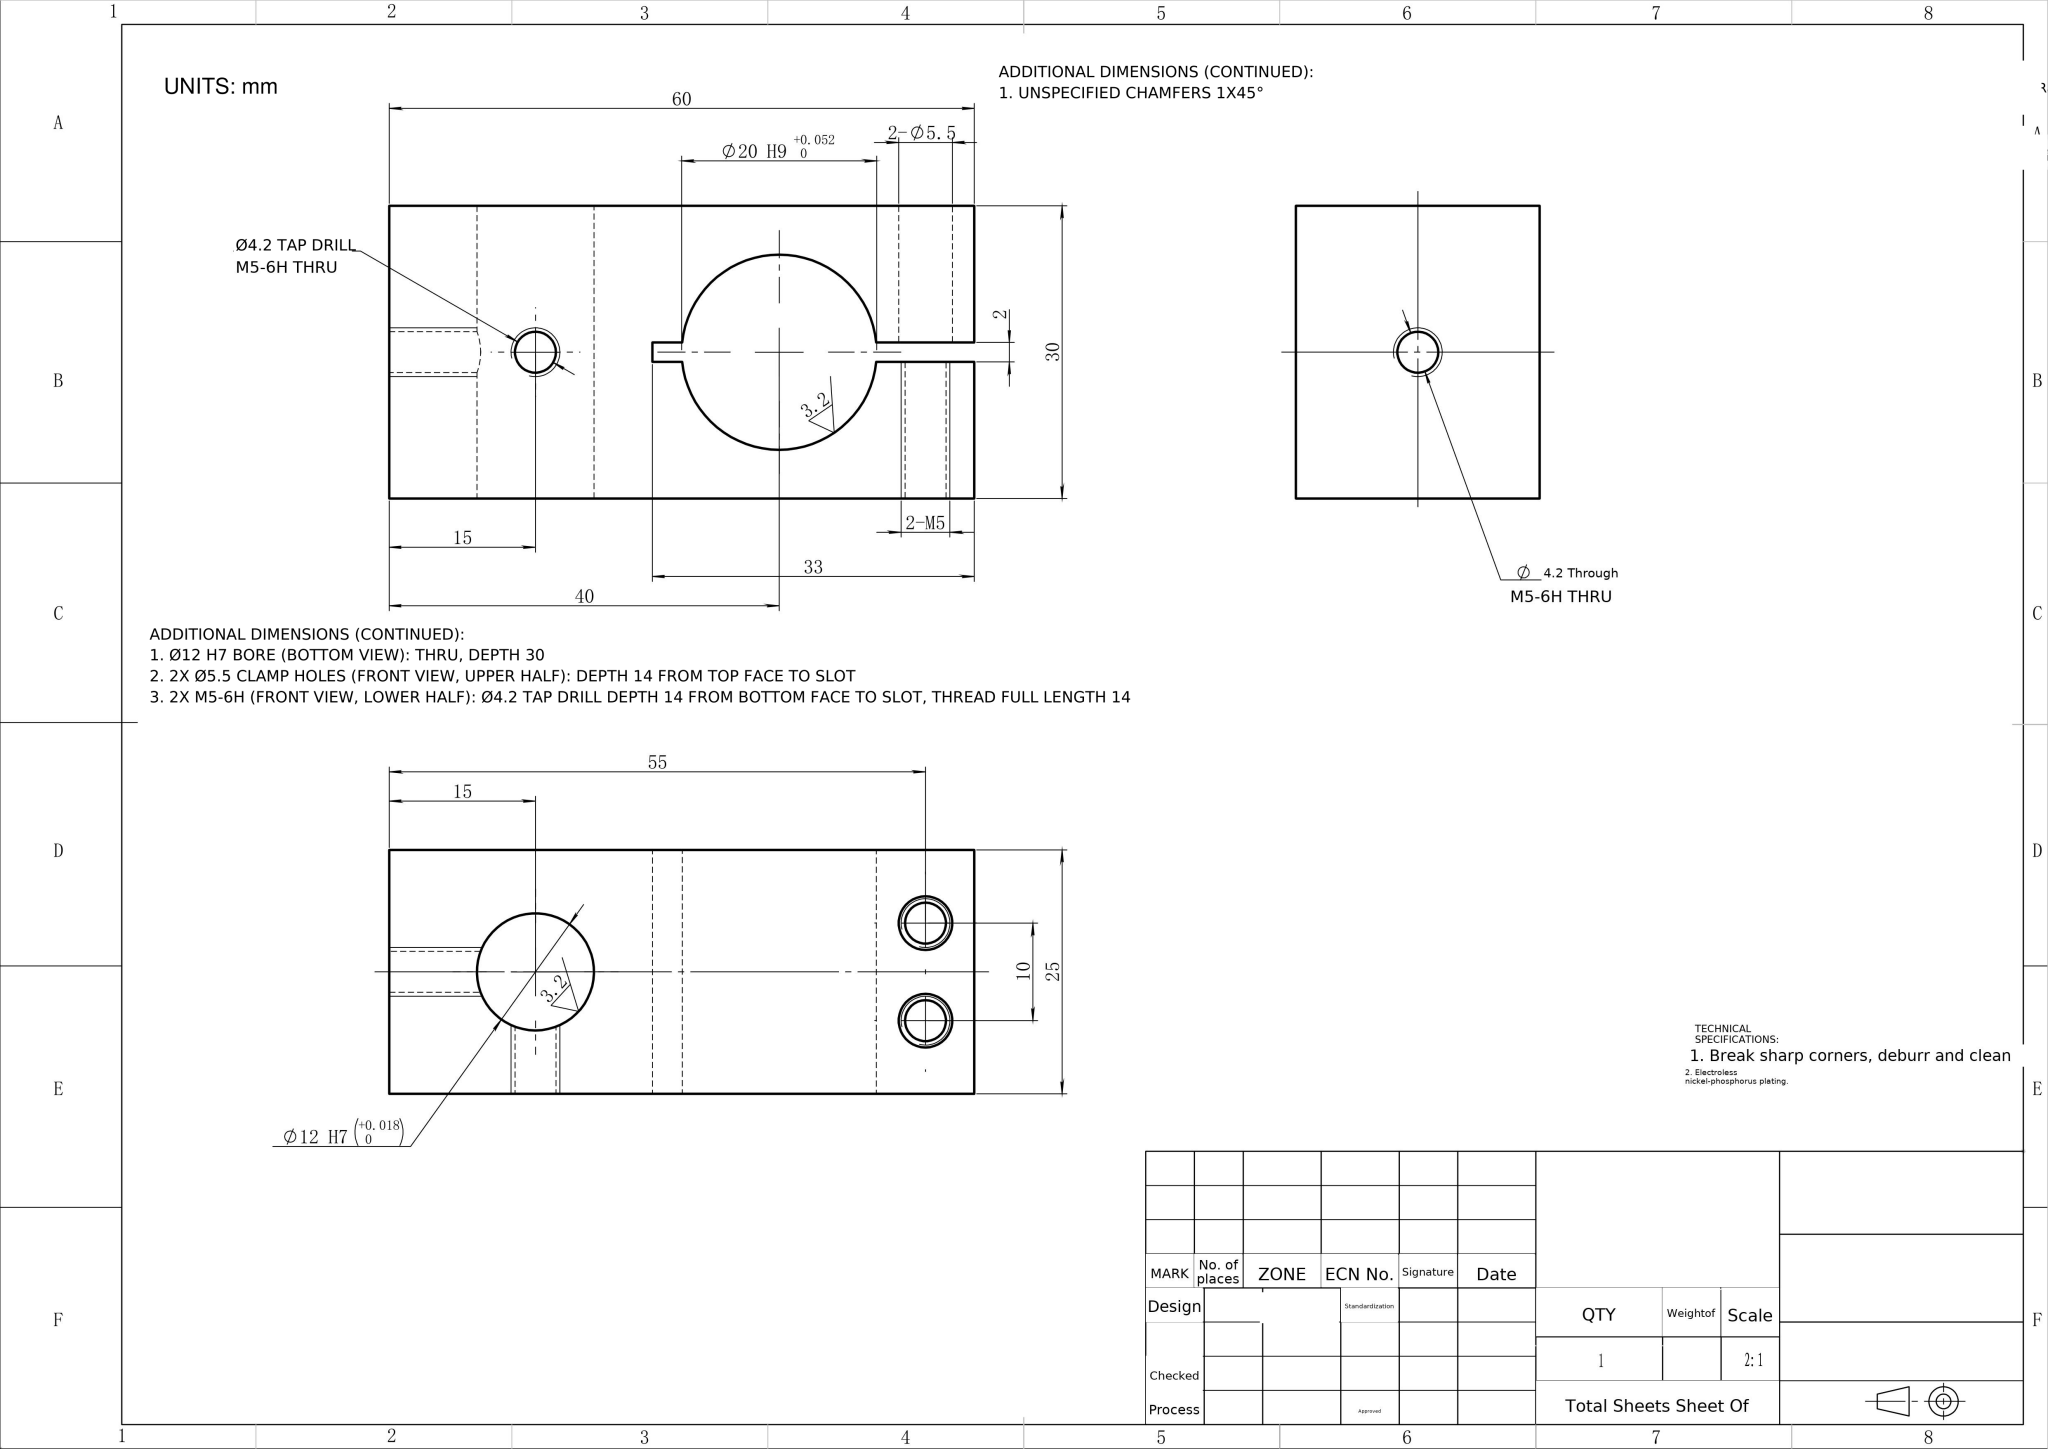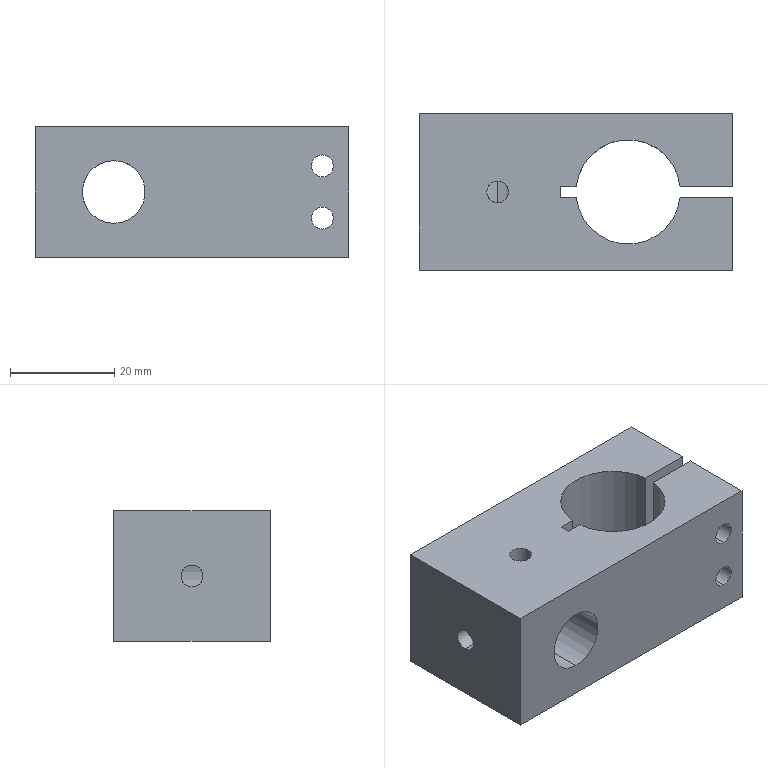Part | NX | mm | 1 solid | 28 faces | box 60 x 30 x 25 mm | volume 31831 mm3 | cylinder 16 | plane 12 | commonest cylinder face diameters 4.2 x8 5.5 x4 12 x2 20 x2